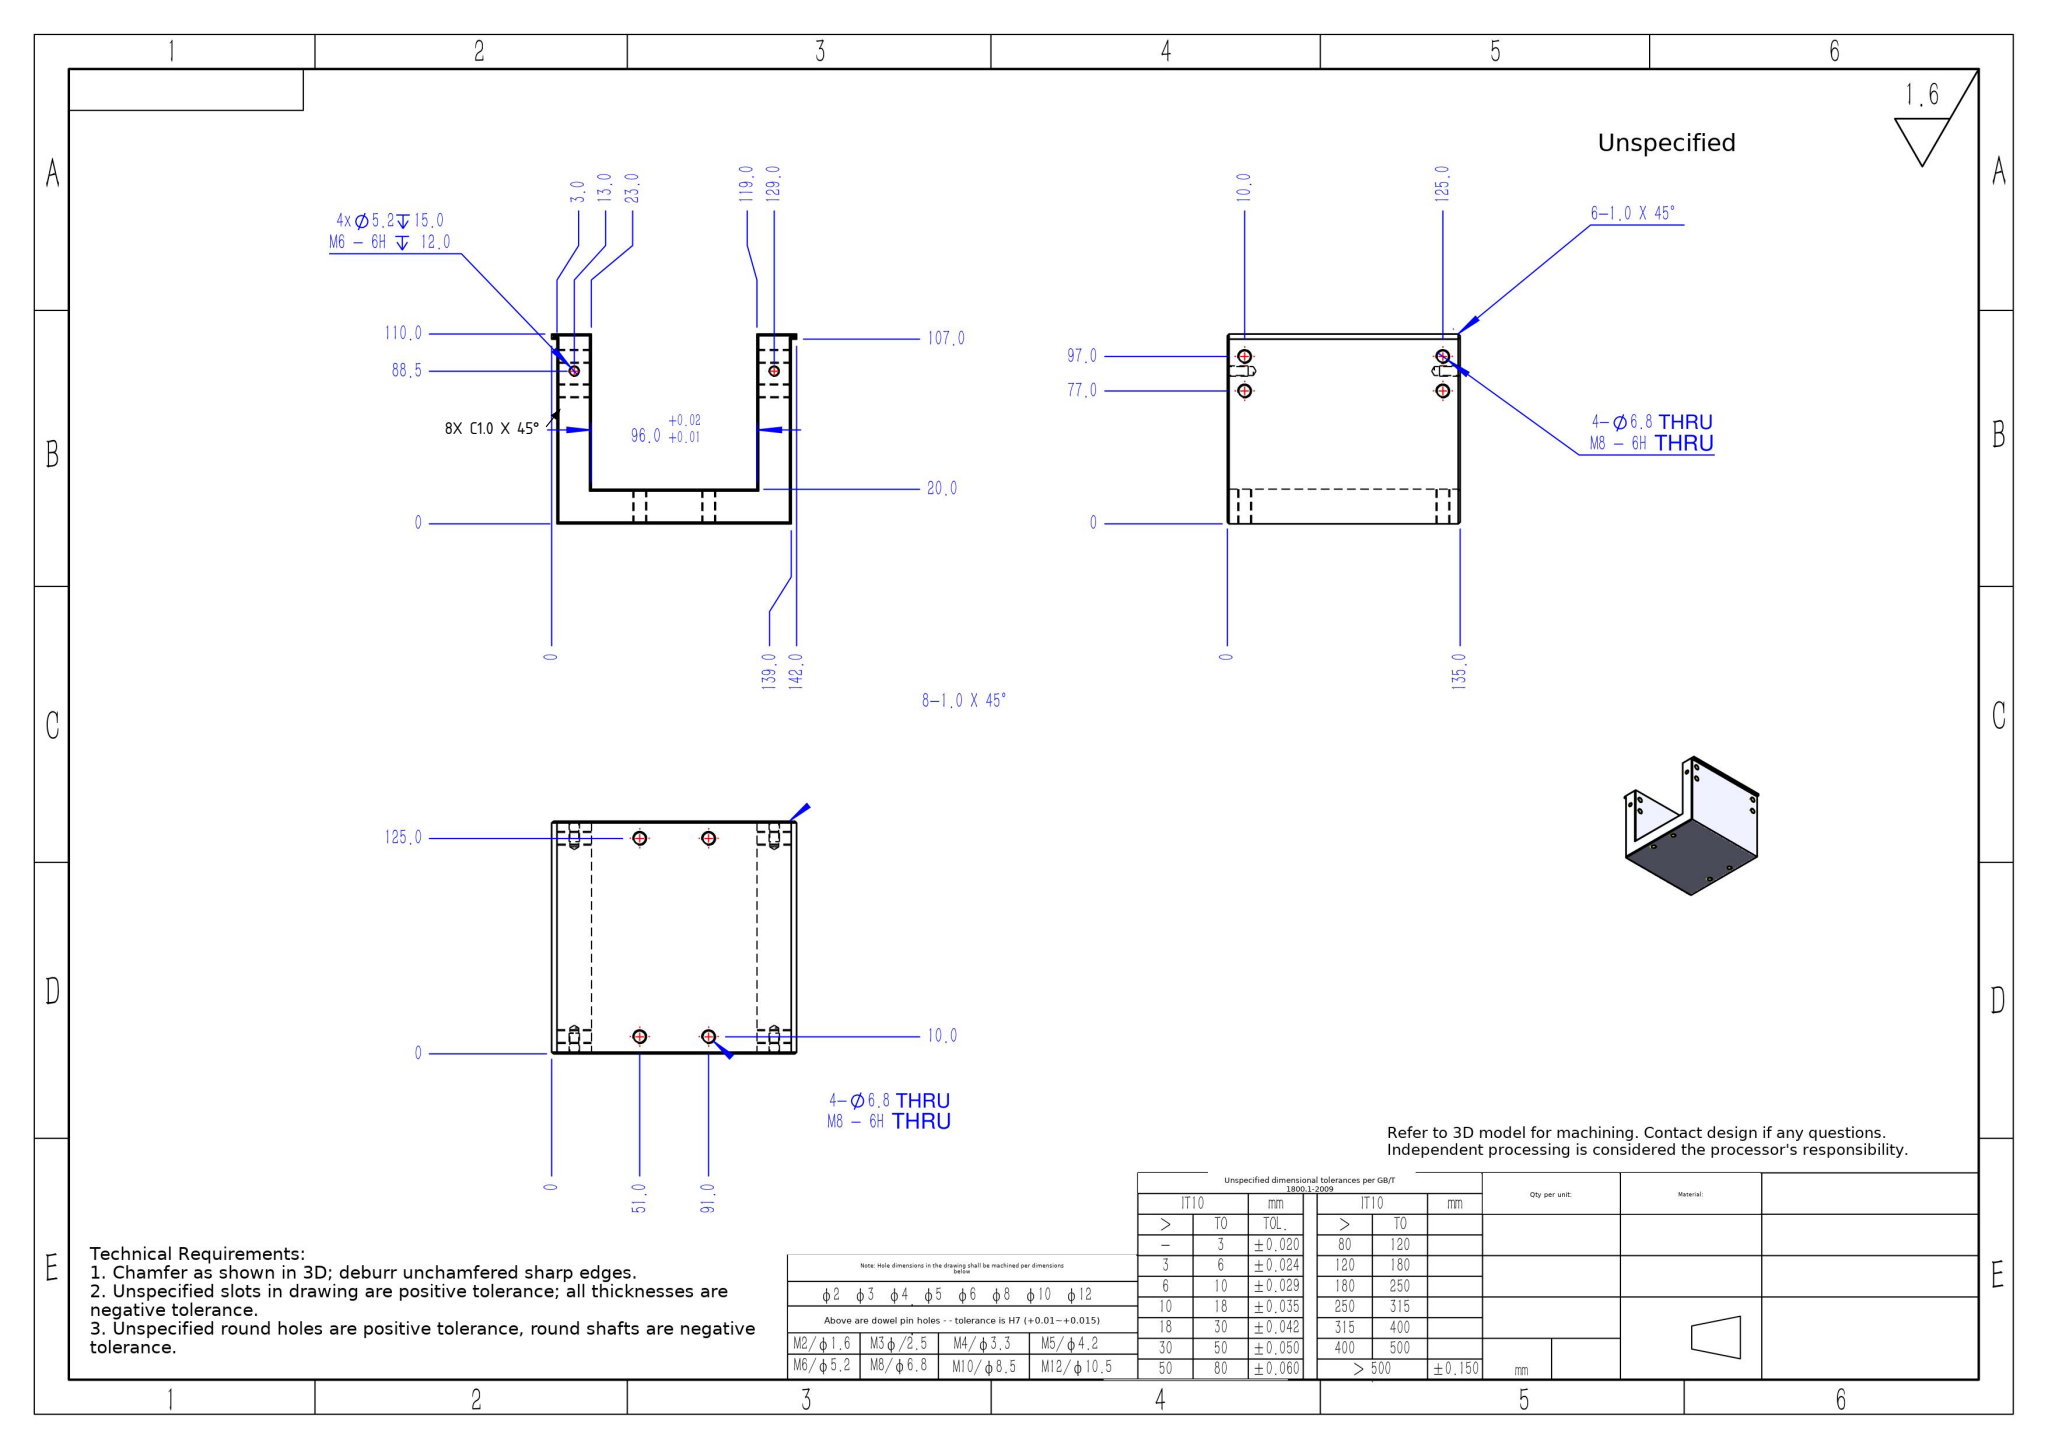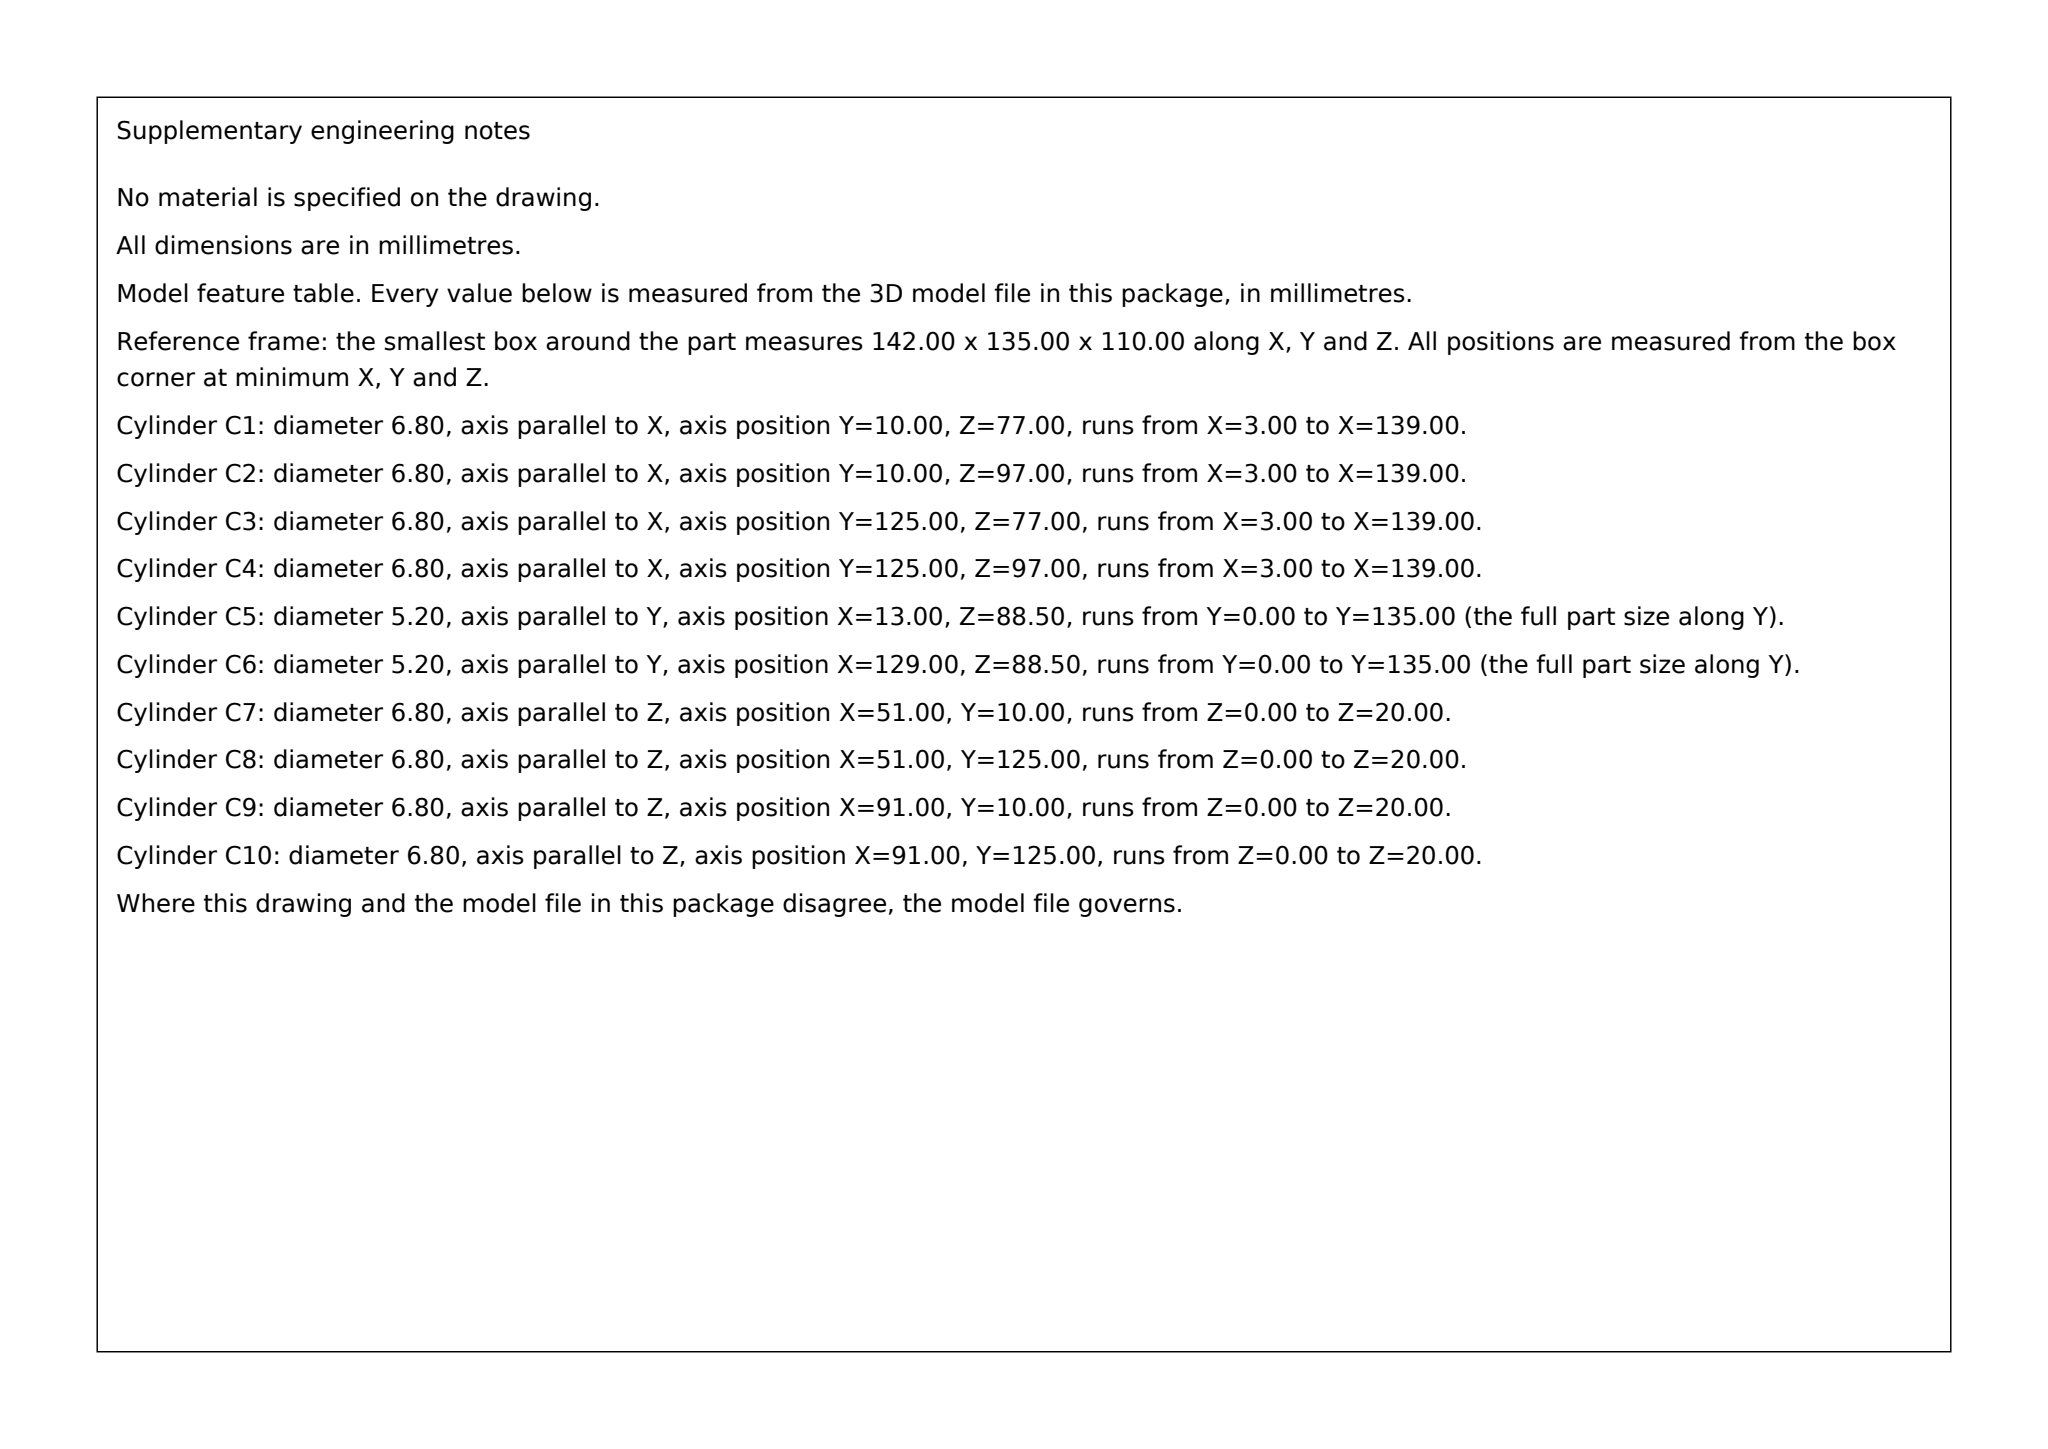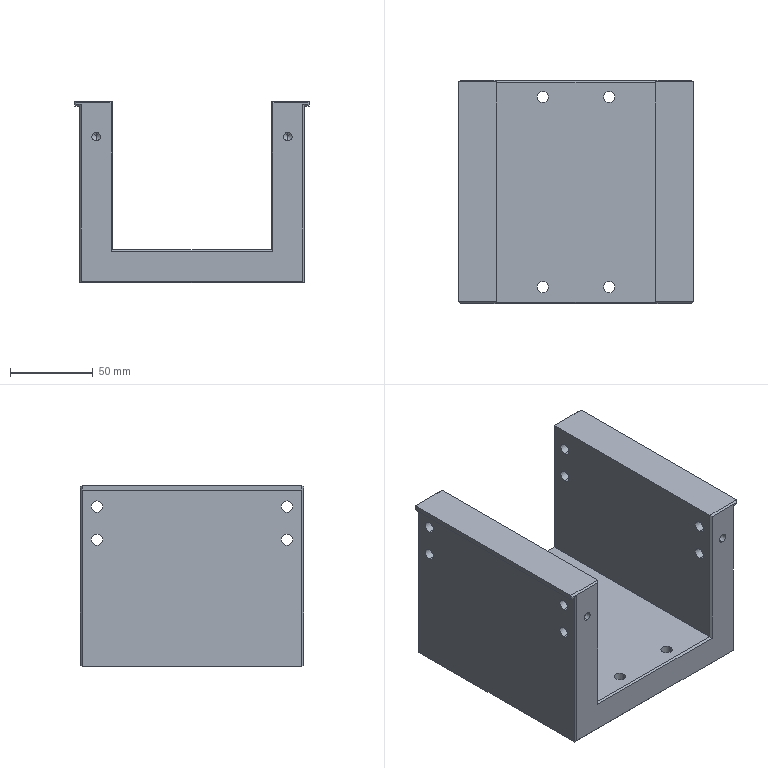Part | SolidWorks | mm | 1 solid | 78 faces | box 142 x 135 x 110 mm | volume 844914 mm3 | plane 38 | cylinder 32 | cone 8 | commonest cylinder face diameters 6.8 x24 5.2 x8
Drawing notes:
8-1.0X45° CHAMFER: VERT EDGES 3, 23, 119, 139 EA SIDE FACE | from the solid: Inclined planes [45,45,90] 1x1 running along Z at corners x=3 & x=139 (z0-108) and x=23 & x=119 (z20-110), each occurring at y=0 and y=135 faces = 8 edges, 1.0 x 45°
build123d program:
from build123d import *

# Parameters (mm, degrees)
SKETCH1_W                  = 142
SKETCH1_H                  = 135
BOSS_EXTRUDE1_DEPTH        = 55
SKETCH2_W                  = 96
SKETCH2_H                  = 90
CUT_EXTRUDE1_DEPTH         = 274
SKETCH3_W                  = 107
SKETCH3_H                  = 135
CUT_EXTRUDE2_DEPTH         = 3
M8_TAPPED_HOLE1_D          = 6.8
CHAMFER1_SIZE              = 1
M8_TAPPED_HOLE2_D          = 6.8
M6_TAPPED_HOLE1_AT_2_COUNT = 2
M6_TAPPED_HOLE1_AT_2_PITCH = 116


with BuildPart() as part:
    # Sketch1 → Boss-Extrude1 (new, symmetric)
    with BuildSketch(Plane.XY):
        Rectangle(SKETCH1_W, SKETCH1_H)
    extrude(amount=BOSS_EXTRUDE1_DEPTH, both=True)

    # Sketch2 → Cut-Extrude1 (cut)
    with BuildSketch(Plane.XZ.offset(67.5)):
        with Locations((0, 10)):
            Rectangle(SKETCH2_W, SKETCH2_H)
    extrude(amount=-CUT_EXTRUDE1_DEPTH, mode=Mode.SUBTRACT)

    # Sketch3 → Cut-Extrude2 (cut)
    with BuildSketch(Plane(origin=(71, 0, 0), x_dir=(0, 0, -1), z_dir=(1, 0, 0))):
        with Locations((1.5, 0)):
            Rectangle(SKETCH3_W, SKETCH3_H)
    cut_extrude2 = extrude(amount=-CUT_EXTRUDE2_DEPTH, mode=Mode.SUBTRACT)

    # Mirror1: Cut-Extrude2 across plane
    add(cut_extrude2.mirror(Plane(origin=(0, 0, 0), x_dir=(0, 0, 1), z_dir=(1, 0, 0))), mode=Mode.SUBTRACT)

    # M8 Tapped Hole1 (through all)
    with Locations(Plane.XY.offset(-35)):
        with Locations((20, 57.5), (-20, 57.5), (-20, -57.5), (20, -57.5)):
            Hole(M8_TAPPED_HOLE1_D / 2)

    # Chamfer1
    chamfer1_edges = [part.edges().sort_by_distance(p)[0] for p in [
        (-59.5, -67.5, 55),
        (-59.5, 67.5, 55),
        (59.5, -67.5, 55),
        (0, 67.5, -35),
        (-48, 67.5, 10),
        (48, 67.5, 10),
        (-48, -67.5, 10),
        (0, -67.5, -35),
        (48, -67.5, 10),
        (0, 67.5, -55),
        (68, -67.5, -1.5),
        (69.5, -67.5, 52),
        (68, 67.5, -1.5),
        (69.5, 67.5, 52),
        (0, -67.5, -55),
        (-69.5, 67.5, 52),
        (-69.5, -67.5, 52),
        (-68, 67.5, -1.5),
        (-68, -67.5, -1.5),
        (59.5, 67.5, 55),
        (71, -67.5, 53.5),
        (-71, -67.5, 53.5),
        (-71, 67.5, 53.5),
        (71, 67.5, 53.5),
    ]]
    chamfer(chamfer1_edges, length=CHAMFER1_SIZE)

    # M8 Tapped Hole2 (through all)
    with Locations(Plane(origin=(68, 0, 0), x_dir=(0, 0, -1), z_dir=(1, 0, 0))):
        with Locations((-42, -57.5), (-22, -57.5), (-22, 57.5), (-42, 57.5)):
            Hole(M8_TAPPED_HOLE2_D / 2)

    # Sketch8 → M6 Tapped Hole1 (revolve, cut)
    with BuildSketch(Plane(origin=(58, -67.5, 33.5), x_dir=(0, 0, -1), z_dir=(1, 0, 0))):
        Polygon((0, 0), (0, 16.562), (2.6, 15), (2.6, 0), align=None)
    m6_tapped_hole1 = revolve(axis=Axis((58, -73.85, 33.5), (0, 1, 0)), mode=Mode.SUBTRACT)

    # M6 Tapped Hole1 at 2: M6 Tapped Hole1 ×2
    with Locations(*[(-i * M6_TAPPED_HOLE1_AT_2_PITCH, 0, 0) for i in range(1, M6_TAPPED_HOLE1_AT_2_COUNT)]):
        add(m6_tapped_hole1, mode=Mode.SUBTRACT)

    # Mirror2: M6 Tapped Hole1 across plane
    add(m6_tapped_hole1.mirror(Plane.ZX), mode=Mode.SUBTRACT)

    # Mirror2 copy 1 sketch → Mirror2 copy 1 (revolve, cut)
    with BuildSketch(Plane(origin=(-58, 67.5, 33.5), x_dir=(0, 0, -1), z_dir=(1, 0, 0))):
        Polygon((0, 0), (0, -16.562), (2.6, -15), (2.6, 0), align=None)
    revolve(axis=Axis((-58, 73.85, 33.5), (0, 1, 0)), mode=Mode.SUBTRACT)


solid = part.part